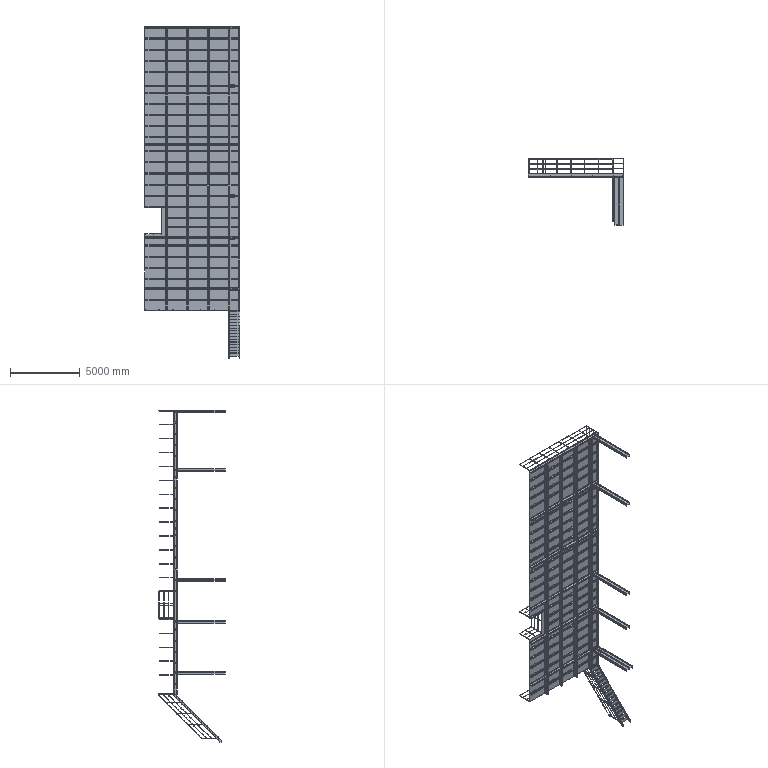Assembly | NX | mm | 46 component files | 228 solids | 3173 faces | box 6880 x 4772.75 x 23866 mm | volume 1941747227 mm3 | plane 2401 | cylinder 734 | spline 36 | other 2 | commonest cylinder face diameters 15 x412 20 x270 32 x42 33.5 x8 22 x2
Bill of materials:
unnamed part 1 | 19 |  | Long straight prismatic member with a wide-flange (H/I) cross-section, rendered as five collinear segments separated by small gaps.
unnamed part 2 | 1 |  | No geometry visible; the supplied image is blank.
unnamed part 3 | 1 |  | Thin, tall rectangular plate or panel with one rectangular notch cut into one long edge, a little below mid-height.
unnamed part 4 | 2 |  | Long straight prismatic member with a wide-flange (H/I) cross-section, rendered as four collinear segments separated by small gaps.
unnamed part 5 | 4 |  | Long straight member with an I cross-section (deep web, narrower flanges), rendered as six collinear segments separated by small gaps.
unnamed part 6 | 1 |  | Long straight continuous member with a channel (C/U) cross-section.
unnamed part 7 | 6 |  | Long straight continuous member with a wide-flange (H/I) cross-section.
unnamed part 8 | 6 |  | Plain flat rectangular plate with uniform thickness.
unnamed part 9 | 6 |  | Straight prismatic member with an H-shaped cross-section made of thin plates with sharp corners. It is relatively short compared with the other beam members.
Mates:
1. touch align | f2 2 face | f1 5 edge
2. touch align | f2 6 face | f1 2 face
3. touch align | f2 6 face | f1 2 face
4. touch align | f2 5 face | f1 1 face
5. touch align | f2 4 face | f1 4 face
6. touch align | f2 1 face | f1 6 face